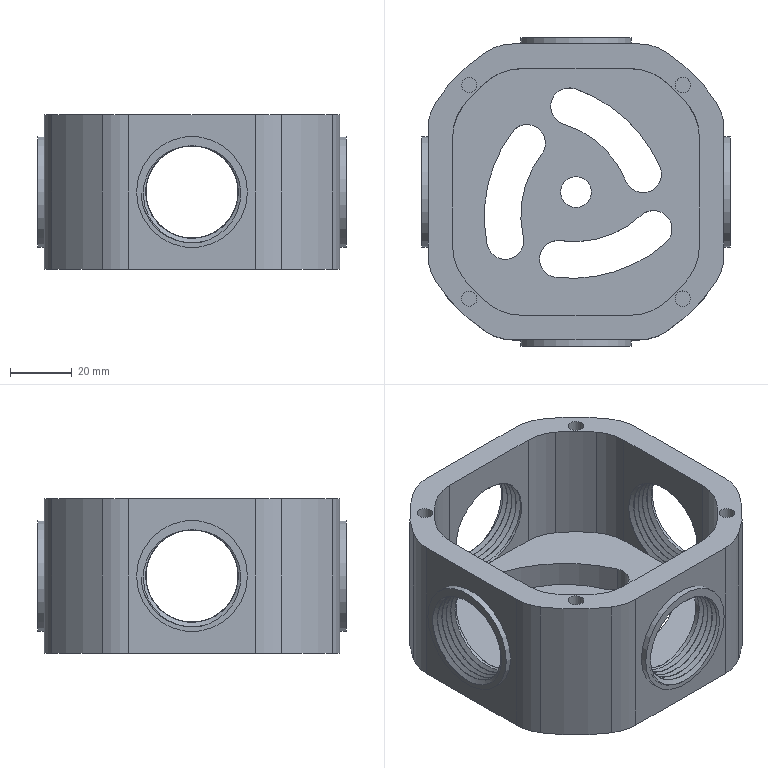Component | NX | BASE | 1 solid | 85 faces | volume 141798 mm3 | cylinder 53 | plane 24 | spline 8 | commonest cylinder face diameters 32 x16 12 x6 30 x4 108 x4 36 x4 92 x4 5 x4 33 x4